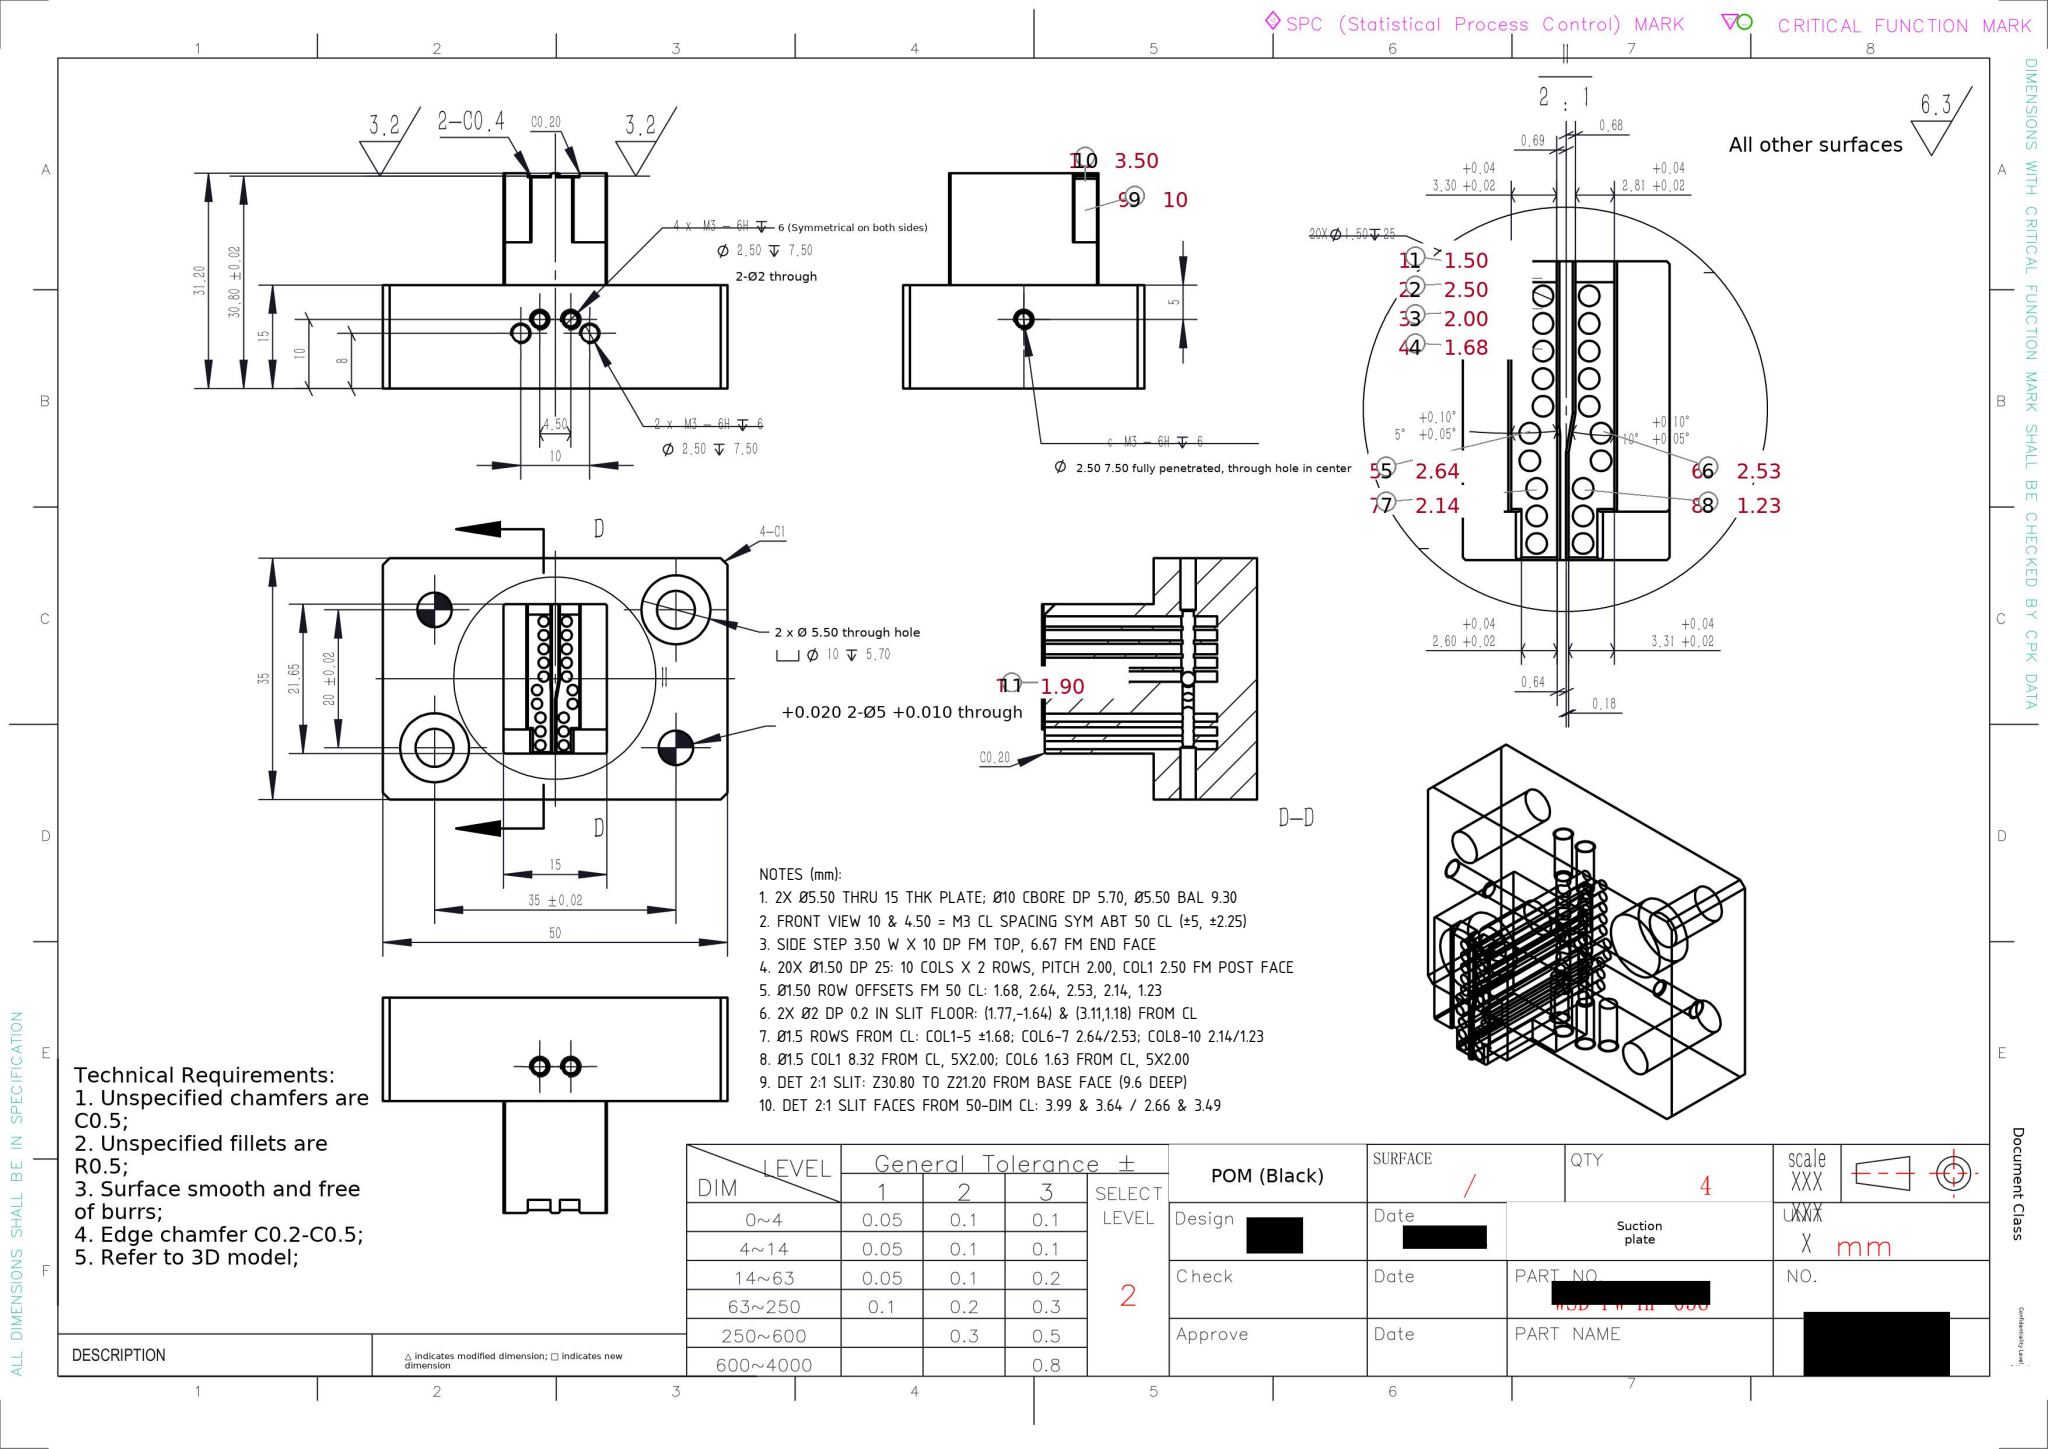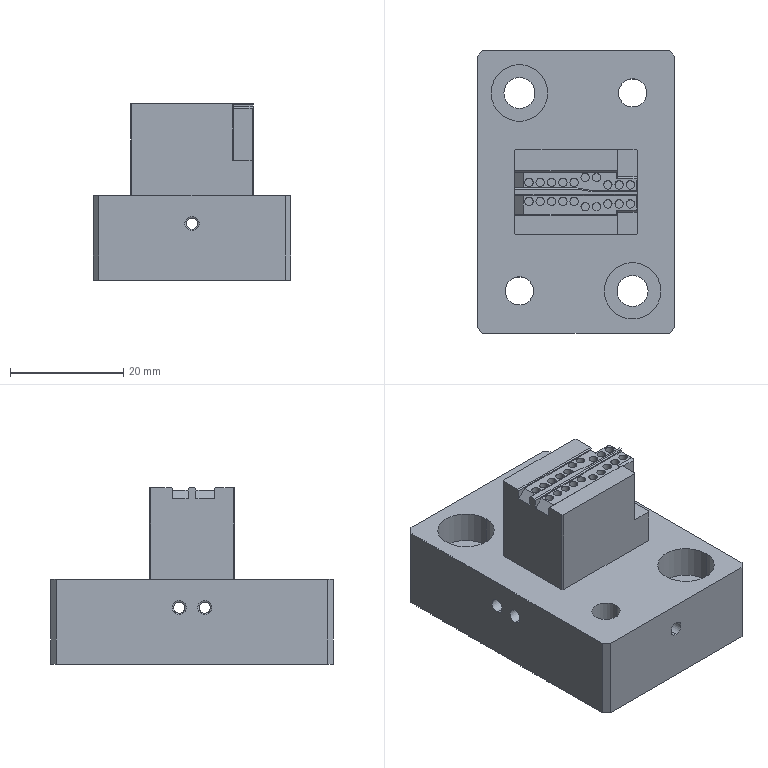Part | SolidWorks | mm | 1 solid | 202 faces | box 35 x 50 x 31.2 mm | volume 27831 mm3 | cylinder 106 | plane 79 | cone 17 | commonest cylinder face diameters 1.5 x62 2.5 x16 2 x16 5 x4 10 x4 5.5 x4
Drawing notes:
2X Ø5.50 THRU 15 THK PLATE; Ø10 CBORE DP 5.70, Ø5.50 BAL 9.30 | from the solid: Ø5.5 z-cyls len 9.30 at (7.5,42.5) & (27.5,7.5); Ø10 z-cyls len 5.70 same axes; plate z 0-15; 9.30+5.70=15
FRONT VIEW 10 & 4.50 = M3 CL SPACING SYM ABT 50 CL (±5, ±2.25) | from the solid: Ø2.5 x-drills at y=20.0 & 30.0 (z8) = 10 apart; y=22.75 & 27.25 (z10) = 4.50 apart; y CL 25.0
SIDE STEP 3.50 W X 10 DP FM TOP, 6.67 FM END FACE | from the solid: x-planes 24.83 & 28.33 (3.50 wide); z 31.2 top to 21.2 (10 deep); 35.0-28.33=6.67
20X Ø1.50 DP 25: 10 COLS X 2 ROWS, PITCH 2.00, COL1 2.50 FM POST FACE | from the solid: Ø1.5 z-holes at x=9.18,11.18,13.18,15.18,17.18,19.13,21.13,23.13,25.13,27.13 (2 per col = 20); post face x-plane 6.68, 9.18-6.68=2.50; depth 25
Ø1.50 ROW OFFSETS FM 50 CL: 1.68, 2.64, 2.53, 2.14, 1.23 | from the solid: y CL = 25.0 (bbox y 50); rows y=23.32/26.68 (1.68), 22.36 (2.64), 27.53 (2.53), 22.86 (2.14), 26.23 (1.23)
2X Ø2 DP 0.2 IN SLIT FLOOR: (1.77,-1.64) & (3.11,1.18) FROM CL | from the solid: cylinders [2.0,"z",[19.27,23.36],0.2] and [2.0,"z",[20.61,26.18],0.2]; bbox 35x50 -> CL at x17.5/y25.0
Ø1.5 ROWS FROM CL: COL1-5 ±1.68; COL6-7 2.64/2.53; COL8-10 2.14/1.23 | from the solid: Ø1.5 y=23.32/26.68 (x9.18-17.18); y=22.36/27.53 (x19.13,21.13); y=22.86/26.23 (x23.13,25.13,27.13); CL y=25.0
Ø1.5 COL1 8.32 FROM CL, 5X2.00; COL6 1.63 FROM CL, 5X2.00 | from the solid: Ø1.5 x = 9.18,11.18,13.18,15.18,17.18 and 19.13,21.13,23.13,25.13,27.13; CL x17.5 (35 dim)
DET 2:1 SLIT: Z30.80 TO Z21.20 FROM BASE FACE (9.6 DEEP) | from the solid: axis planes z=30.8 (2) and z=21.2 (2); Ø1.5 ↧25 runs 30.8 to 5.8
DET 2:1 SLIT FACES FROM 50-DIM CL: 3.99 & 3.64 / 2.66 & 3.49 | from the solid: y planes 21.01, 21.36, 27.66, 28.49 vs CL y=25.0 of 50 bbox